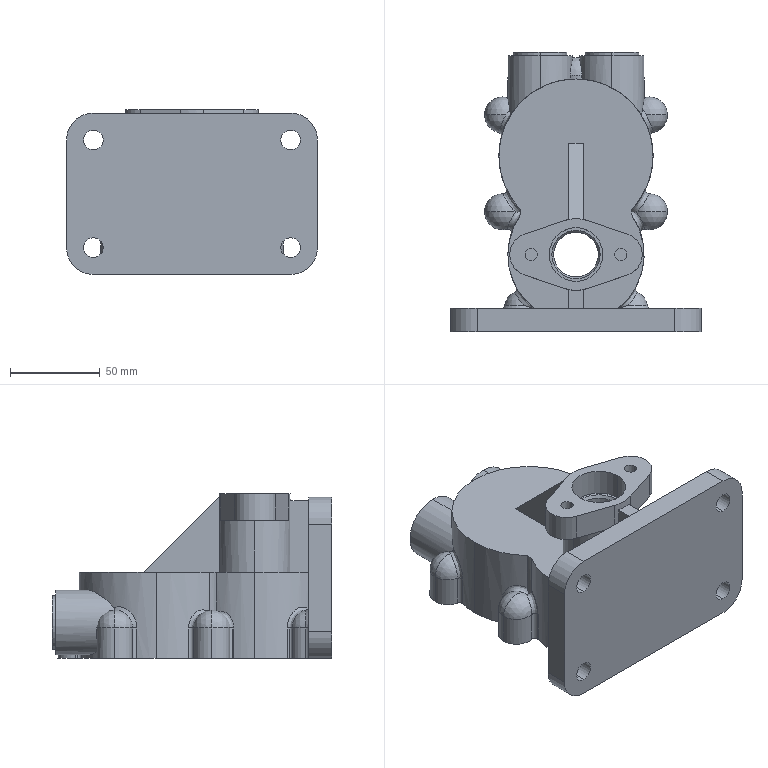Component | SolidWorks | PumpBody-1 | 1 solid | 197 faces | volume 437963 mm3 | cylinder 109 | cone 34 | plane 32 | sphere 12 | spline 8 | torus 2 | commonest cylinder face diameters 4 x18 6.8 x18 20 x14 11 x12 24 x11 30 x10 86 x5 16.5 x4